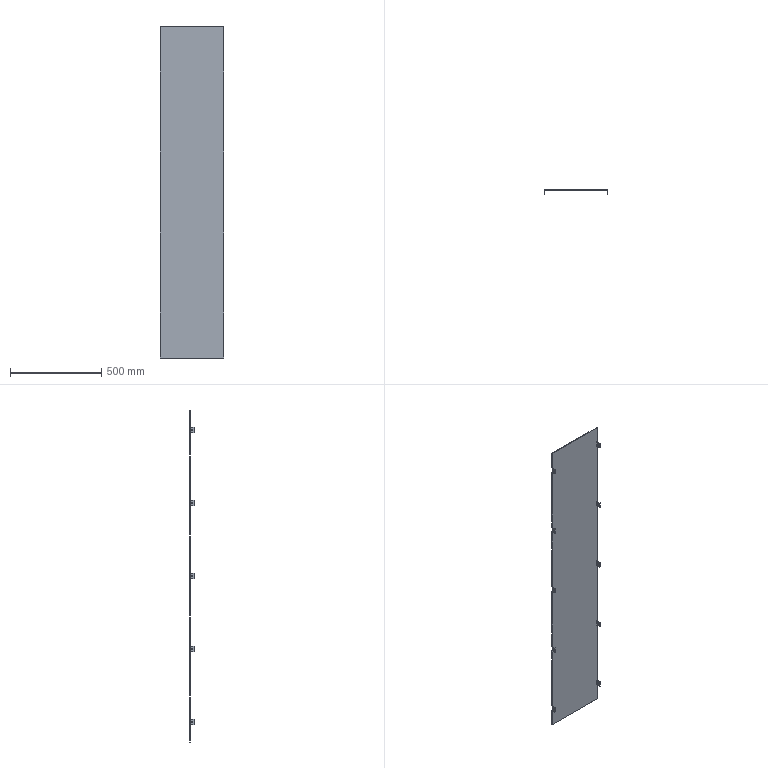Component | SolidWorks | SidePartition(Item25)-3 | 1 solid | 196 faces | volume 1285506 mm3 | plane 146 | cylinder 50 | commonest cylinder face diameters 6.5 x30 6 x10 2 x10 | material Plain Carbon Steel